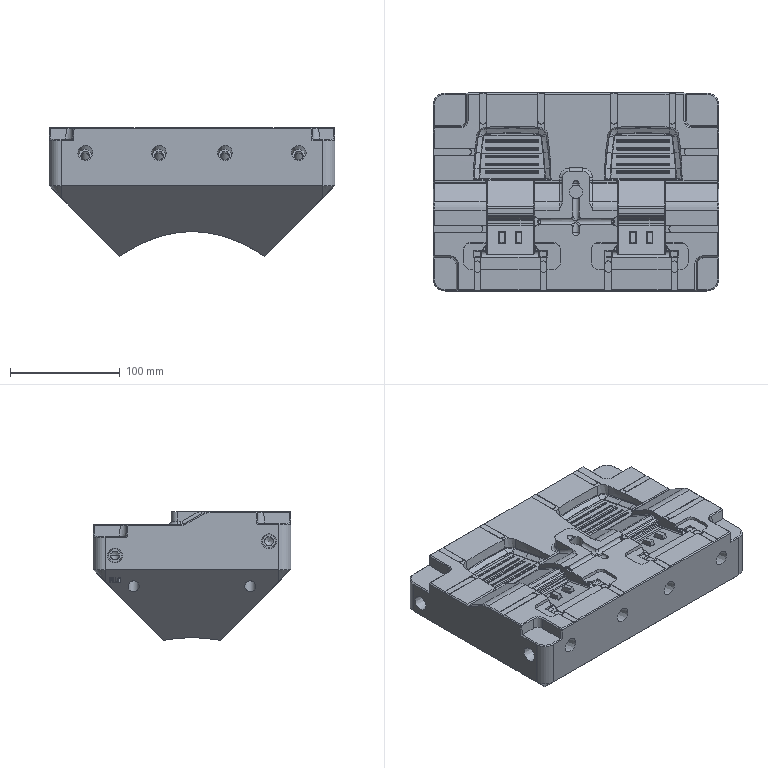CAM job | NX | mm | 3-axis | 1 set-up | 2 operations | part box 260 x 180 x 117.19
set-up 1
1. Volume Based 2.5D Milling | Mill Mill5 D4 | FLOOR_WALL_1 | path 4344.008 mm | 12.324 min
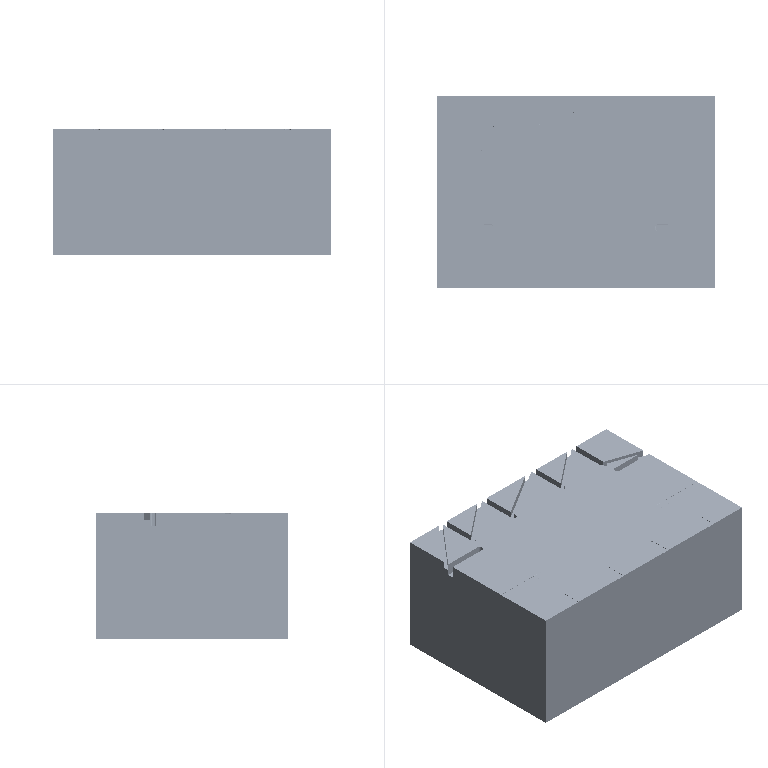2. Volume Based 2.5D Milling | Mill Mill5 D4 | FLOOR_WALL_1_COPY | path 1254.185 mm | 3.621 min